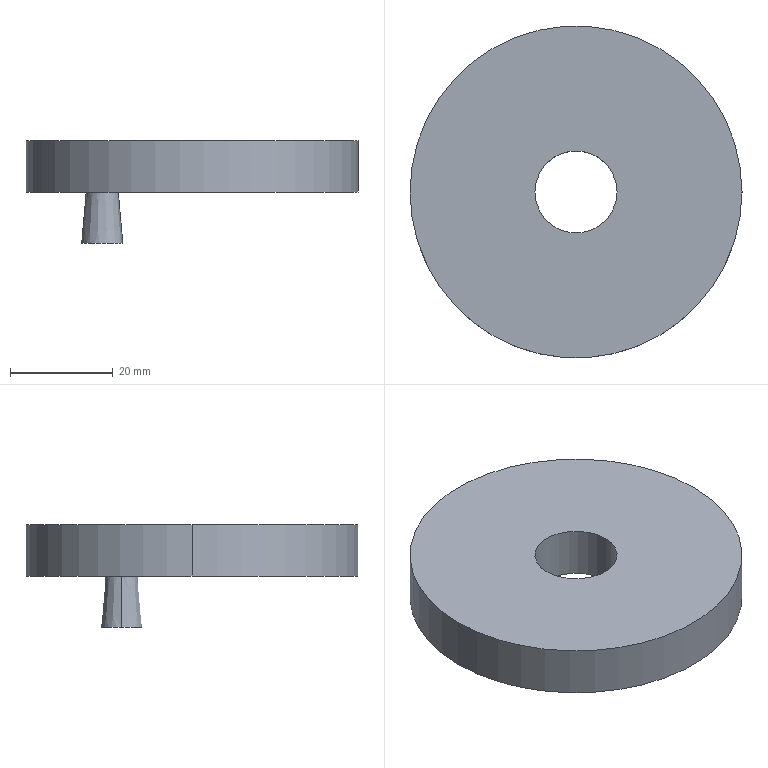Component | SolidWorks | RockerArm-1 | 1 solid | 9 faces | box 64.66 x 64.66 x 20 mm | volume 31223 mm3 | cylinder 4 | plane 3 | cone 2 | commonest cylinder face diameters 16 x2 64.655 x2
build123d program:
from build123d import *

# Parameters (mm, degrees)
SKETCH1_R           = 32.328
SKETCH1_R_2         = 8
BOSS_EXTRUDE1_DEPTH = 10
SKETCH2_R           = 3.13
BOSS_EXTRUDE2_DEPTH = 10
BOSS_EXTRUDE2_DRAFT = -5


with BuildPart() as part:
    # Sketch1 → Boss-Extrude1 (new body)
    with BuildSketch(Plane.XY):
        with Locations((0, -208.707)):
            Circle(SKETCH1_R)
        with Locations((0, -208.707)):
            Circle(SKETCH1_R_2, mode=Mode.SUBTRACT)
    extrude(amount=-BOSS_EXTRUDE1_DEPTH)


with BuildPart() as boss_extrude2_tool:
    # Sketch2 → Boss-Extrude2 (with draft: the straight prism first)
    with BuildSketch(Plane.XY):
        with Locations((17.482, -194.977)):
            Circle(SKETCH2_R)
    extrude(amount=BOSS_EXTRUDE2_DEPTH)
    # Boss-Extrude2: the draft: its side faces are tilted about the plane it starts from
    boss_extrude2_sides = [boss_extrude2_tool.faces().sort_by_distance(p)[0] for p in [
        (14.352, -194.977, 5),
    ]]
    draft(boss_extrude2_sides, Plane.XY, BOSS_EXTRUDE2_DRAFT)


with BuildPart() as part_1:
    add(part.part)

    # Boss-Extrude2: add boss_extrude2_tool
    add(boss_extrude2_tool.part)


solid = part_1.part

# Placed as in the assembly
solid = solid.moved(Location((0, 0, -657.565), (-180, 0, 180)))
STEP:
#1=COLOUR_RGB('',0.7922,0.8196,0.9333);
#2=FILL_AREA_STYLE_COLOUR('',#1);
#3=FILL_AREA_STYLE('',(#2));
#4=SURFACE_STYLE_FILL_AREA(#3);
#5=SURFACE_SIDE_STYLE('',(#4));
#6=SURFACE_STYLE_USAGE(.BOTH.,#5);
#7=PRESENTATION_STYLE_ASSIGNMENT((#6));
#8=CARTESIAN_POINT('',(-0.8115,-7.676,-25.888));
#9=VERTEX_POINT('',#8);
#10=CARTESIAN_POINT('',(-0.5651,-7.676,-25.888));
#11=VERTEX_POINT('',#10);
#12=CARTESIAN_POINT('',(-0.6883,-7.676,-25.888));
#13=DIRECTION('',(0.,0.,-1.));
#14=DIRECTION('',(-1.,0.,0.));
#15=AXIS2_PLACEMENT_3D('',#12,#13,#14);
#16=CIRCLE('',#15,0.1232);
#17=EDGE_CURVE('',#9,#11,#16,.T.);
#18=ORIENTED_EDGE('',*,*,#17,.T.);
#19=CARTESIAN_POINT('',(-0.5306,-7.676,-26.282));
#20=VERTEX_POINT('',#19);
#21=CARTESIAN_POINT('',(-0.5651,-7.676,-25.888));
#22=DIRECTION('',(0.08716,0.,-0.9962));
#23=VECTOR('',#22,39.37);
#24=LINE('',#21,#23);
#25=EDGE_CURVE('',#11,#20,#24,.T.);
#26=ORIENTED_EDGE('',*,*,#25,.T.);
#27=CARTESIAN_POINT('',(-0.8459,-7.676,-26.282));
#28=VERTEX_POINT('',#27);
#29=CARTESIAN_POINT('',(-0.6883,-7.676,-26.282));
#30=DIRECTION('',(0.,0.,-1.));
#31=DIRECTION('',(-1.,0.,0.));
#32=AXIS2_PLACEMENT_3D('',#29,#30,#31);
#33=CIRCLE('',#32,0.1577);
#34=EDGE_CURVE('',#28,#20,#33,.T.);
#35=ORIENTED_EDGE('',*,*,#34,.F.);
#36=CARTESIAN_POINT('',(-0.8115,-7.676,-25.888));
#37=DIRECTION('',(-0.08716,0.,-0.9962));
#38=VECTOR('',#37,39.37);
#39=LINE('',#36,#38);
#40=EDGE_CURVE('',#9,#28,#39,.T.);
#41=ORIENTED_EDGE('',*,*,#40,.F.);
#42=EDGE_LOOP('',(#18,#26,#35,#41));
#43=FACE_OUTER_BOUND('',#42,.T.);
#44=CARTESIAN_POINT('',(-0.6883,-7.676,-25.888));
#45=DIRECTION('',(0.,0.,-1.));
#46=DIRECTION('',(-1.,0.,0.));
#47=AXIS2_PLACEMENT_3D('',#44,#45,#46);
#48=CONICAL_SURFACE('',#47,0.1232,0.08727);
#49=ADVANCED_FACE('',(#43),#48,.T.);
#50=CARTESIAN_POINT('',(0.315,-8.217,-25.495));
#51=VERTEX_POINT('',#50);
#52=CARTESIAN_POINT('',(-0.315,-8.217,-25.495));
#53=VERTEX_POINT('',#52);
#54=CARTESIAN_POINT('',(0.,-8.217,-25.495));
#55=DIRECTION('',(0.,0.,-1.));
#56=DIRECTION('',(-1.,0.,0.));
#57=AXIS2_PLACEMENT_3D('',#54,#55,#56);
#58=CIRCLE('',#57,0.315);
#59=EDGE_CURVE('',#51,#53,#58,.T.);
#60=ORIENTED_EDGE('',*,*,#59,.F.);
#61=CARTESIAN_POINT('',(0.315,-8.217,-25.888));
#62=VERTEX_POINT('',#61);
#63=CARTESIAN_POINT('',(0.315,-8.217,-25.495));
#64=DIRECTION('',(0.,0.,-1.));
#65=VECTOR('',#64,39.37);
#66=LINE('',#63,#65);
#67=EDGE_CURVE('',#51,#62,#66,.T.);
#68=ORIENTED_EDGE('',*,*,#67,.T.);
#69=CARTESIAN_POINT('',(-0.315,-8.217,-25.888));
#70=VERTEX_POINT('',#69);
#71=CARTESIAN_POINT('',(0.,-8.217,-25.888));
#72=DIRECTION('',(0.,0.,-1.));
#73=DIRECTION('',(-1.,0.,0.));
#74=AXIS2_PLACEMENT_3D('',#71,#72,#73);
#75=CIRCLE('',#74,0.315);
#76=EDGE_CURVE('',#62,#70,#75,.T.);
#77=ORIENTED_EDGE('',*,*,#76,.T.);
#78=CARTESIAN_POINT('',(-0.315,-8.217,-25.495));
#79=DIRECTION('',(0.,0.,-1.));
#80=VECTOR('',#79,39.37);
#81=LINE('',#78,#80);
#82=EDGE_CURVE('',#53,#70,#81,.T.);
#83=ORIENTED_EDGE('',*,*,#82,.F.);
#84=EDGE_LOOP('',(#60,#68,#77,#83));
#85=FACE_OUTER_BOUND('',#84,.T.);
#86=CARTESIAN_POINT('',(0.,-8.217,-25.495));
#87=DIRECTION('',(0.,0.,-1.));
#88=DIRECTION('',(-1.,0.,0.));
#89=AXIS2_PLACEMENT_3D('',#86,#87,#88);
#90=CYLINDRICAL_SURFACE('',#89,0.315);
#91=ADVANCED_FACE('',(#85),#90,.F.);
#92=CARTESIAN_POINT('',(-1.273,-8.217,-25.495));
#93=VERTEX_POINT('',#92);
#94=CARTESIAN_POINT('',(1.273,-8.217,-25.495));
#95=VERTEX_POINT('',#94);
#96=CARTESIAN_POINT('',(0.,-8.217,-25.495));
#97=DIRECTION('',(0.,0.,-1.));
#98=DIRECTION('',(-1.,0.,0.));
#99=AXIS2_PLACEMENT_3D('',#96,#97,#98);
#100=CIRCLE('',#99,1.273);
#101=EDGE_CURVE('',#93,#95,#100,.T.);
#102=ORIENTED_EDGE('',*,*,#101,.T.);
#103=CARTESIAN_POINT('',(1.273,-8.217,-25.888));
#104=VERTEX_POINT('',#103);
#105=CARTESIAN_POINT('',(1.273,-8.217,-25.495));
#106=DIRECTION('',(0.,0.,-1.));
#107=VECTOR('',#106,39.37);
#108=LINE('',#105,#107);
#109=EDGE_CURVE('',#95,#104,#108,.T.);
#110=ORIENTED_EDGE('',*,*,#109,.T.);
#111=CARTESIAN_POINT('',(-1.273,-8.217,-25.888));
#112=VERTEX_POINT('',#111);
#113=CARTESIAN_POINT('',(0.,-8.217,-25.888));
#114=DIRECTION('',(0.,0.,-1.));
#115=DIRECTION('',(-1.,0.,0.));
#116=AXIS2_PLACEMENT_3D('',#113,#114,#115);
#117=CIRCLE('',#116,1.273);
#118=EDGE_CURVE('',#112,#104,#117,.T.);
#119=ORIENTED_EDGE('',*,*,#118,.F.);
#120=CARTESIAN_POINT('',(-1.273,-8.217,-25.495));
#121=DIRECTION('',(0.,0.,-1.));
#122=VECTOR('',#121,39.37);
#123=LINE('',#120,#122);
#124=EDGE_CURVE('',#93,#112,#123,.T.);
#125=ORIENTED_EDGE('',*,*,#124,.F.);
#126=EDGE_LOOP('',(#102,#110,#119,#125));
#127=FACE_OUTER_BOUND('',#126,.T.);
#128=CARTESIAN_POINT('',(0.,-8.217,-25.495));
#129=DIRECTION('',(0.,0.,-1.));
#130=DIRECTION('',(-1.,0.,0.));
#131=AXIS2_PLACEMENT_3D('',#128,#129,#130);
#132=CYLINDRICAL_SURFACE('',#131,1.273);
#133=ADVANCED_FACE('',(#127),#132,.T.);
#134=ORIENTED_EDGE('',*,*,#109,.F.);
#135=CARTESIAN_POINT('',(0.,-8.217,-25.495));
#136=DIRECTION('',(0.,0.,-1.));
#137=DIRECTION('',(-1.,0.,0.));
#138=AXIS2_PLACEMENT_3D('',#135,#136,#137);
#139=CIRCLE('',#138,1.273);
#140=EDGE_CURVE('',#95,#93,#139,.T.);
#141=ORIENTED_EDGE('',*,*,#140,.T.);
#142=ORIENTED_EDGE('',*,*,#124,.T.);
#143=CARTESIAN_POINT('',(0.,-8.217,-25.888));
#144=DIRECTION('',(0.,0.,-1.));
#145=DIRECTION('',(-1.,0.,0.));
#146=AXIS2_PLACEMENT_3D('',#143,#144,#145);
#147=CIRCLE('',#146,1.273);
#148=EDGE_CURVE('',#104,#112,#147,.T.);
#149=ORIENTED_EDGE('',*,*,#148,.F.);
#150=EDGE_LOOP('',(#134,#141,#142,#149));
#151=FACE_OUTER_BOUND('',#150,.T.);
#152=CARTESIAN_POINT('',(0.,-8.217,-25.495));
#153=DIRECTION('',(0.,0.,-1.));
#154=DIRECTION('',(-1.,0.,0.));
#155=AXIS2_PLACEMENT_3D('',#152,#153,#154);
#156=CYLINDRICAL_SURFACE('',#155,1.273);
#157=ADVANCED_FACE('',(#151),#156,.T.);
#158=CARTESIAN_POINT('',(0.,-8.217,-25.495));
#159=DIRECTION('',(0.,0.,-1.));
#160=DIRECTION('',(-1.,0.,0.));
#161=AXIS2_PLACEMENT_3D('',#158,#159,#160);
#162=CIRCLE('',#161,0.315);
#163=EDGE_CURVE('',#53,#51,#162,.T.);
#164=ORIENTED_EDGE('',*,*,#163,.T.);
#165=ORIENTED_EDGE('',*,*,#59,.T.);
#166=EDGE_LOOP('',(#164,#165));
#167=FACE_BOUND('',#166,.T.);
#168=ORIENTED_EDGE('',*,*,#101,.F.);
#169=ORIENTED_EDGE('',*,*,#140,.F.);
#170=EDGE_LOOP('',(#168,#169));
#171=FACE_OUTER_BOUND('',#170,.T.);
#172=CARTESIAN_POINT('',(0.,-8.217,-25.495));
#173=DIRECTION('',(0.,0.,-1.));
#174=DIRECTION('',(-1.,0.,0.));
#175=AXIS2_PLACEMENT_3D('',#172,#173,#174);
#176=PLANE('',#175);
#177=ADVANCED_FACE('',(#167,#171),#176,.F.);
#178=ORIENTED_EDGE('',*,*,#17,.F.);
#179=CARTESIAN_POINT('',(-0.6883,-7.676,-25.888));
#180=DIRECTION('',(0.,0.,-1.));
#181=DIRECTION('',(-1.,0.,0.));
#182=AXIS2_PLACEMENT_3D('',#179,#180,#181);
#183=CIRCLE('',#182,0.1232);
#184=EDGE_CURVE('',#11,#9,#183,.T.);
#185=ORIENTED_EDGE('',*,*,#184,.F.);
#186=EDGE_LOOP('',(#178,#185));
#187=FACE_BOUND('',#186,.T.);
#188=CARTESIAN_POINT('',(0.,-8.217,-25.888));
#189=DIRECTION('',(0.,0.,-1.));
#190=DIRECTION('',(-1.,0.,0.));
#191=AXIS2_PLACEMENT_3D('',#188,#189,#190);
#192=CIRCLE('',#191,0.315);
#193=EDGE_CURVE('',#70,#62,#192,.T.);
#194=ORIENTED_EDGE('',*,*,#193,.F.);
#195=ORIENTED_EDGE('',*,*,#76,.F.);
#196=EDGE_LOOP('',(#194,#195));
#197=FACE_BOUND('',#196,.T.);
#198=ORIENTED_EDGE('',*,*,#118,.T.);
#199=ORIENTED_EDGE('',*,*,#148,.T.);
#200=EDGE_LOOP('',(#198,#199));
#201=FACE_OUTER_BOUND('',#200,.T.);
#202=CARTESIAN_POINT('',(0.,-8.217,-25.888));
#203=DIRECTION('',(0.,0.,-1.));
#204=DIRECTION('',(-1.,0.,0.));
#205=AXIS2_PLACEMENT_3D('',#202,#203,#204);
#206=PLANE('',#205);
#207=ADVANCED_FACE('',(#187,#197,#201),#206,.T.);
#208=ORIENTED_EDGE('',*,*,#67,.F.);
#209=ORIENTED_EDGE('',*,*,#163,.F.);
#210=ORIENTED_EDGE('',*,*,#82,.T.);
#211=ORIENTED_EDGE('',*,*,#193,.T.);
#212=EDGE_LOOP('',(#208,#209,#210,#211));
#213=FACE_OUTER_BOUND('',#212,.T.);
#214=CARTESIAN_POINT('',(0.,-8.217,-25.495));
#215=DIRECTION('',(0.,0.,-1.));
#216=DIRECTION('',(-1.,0.,0.));
#217=AXIS2_PLACEMENT_3D('',#214,#215,#216);
#218=CYLINDRICAL_SURFACE('',#217,0.315);
#219=ADVANCED_FACE('',(#213),#218,.F.);
#220=ORIENTED_EDGE('',*,*,#25,.F.);
#221=ORIENTED_EDGE('',*,*,#184,.T.);
#222=ORIENTED_EDGE('',*,*,#40,.T.);
#223=CARTESIAN_POINT('',(-0.6883,-7.676,-26.282));
#224=DIRECTION('',(0.,0.,-1.));
#225=DIRECTION('',(-1.,0.,0.));
#226=AXIS2_PLACEMENT_3D('',#223,#224,#225);
#227=CIRCLE('',#226,0.1577);
#228=EDGE_CURVE('',#20,#28,#227,.T.);
#229=ORIENTED_EDGE('',*,*,#228,.F.);
#230=EDGE_LOOP('',(#220,#221,#222,#229));
#231=FACE_OUTER_BOUND('',#230,.T.);
#232=CARTESIAN_POINT('',(-0.6883,-7.676,-25.888));
#233=DIRECTION('',(0.,0.,-1.));
#234=DIRECTION('',(-1.,0.,0.));
#235=AXIS2_PLACEMENT_3D('',#232,#233,#234);
#236=CONICAL_SURFACE('',#235,0.1232,0.08727);
#237=ADVANCED_FACE('',(#231),#236,.T.);
#238=ORIENTED_EDGE('',*,*,#34,.T.);
#239=ORIENTED_EDGE('',*,*,#228,.T.);
#240=EDGE_LOOP('',(#238,#239));
#241=FACE_OUTER_BOUND('',#240,.T.);
#242=CARTESIAN_POINT('',(-0.6883,-7.676,-26.282));
#243=DIRECTION('',(0.,0.,-1.));
#244=DIRECTION('',(-1.,0.,0.));
#245=AXIS2_PLACEMENT_3D('',#242,#243,#244);
#246=PLANE('',#245);
#247=ADVANCED_FACE('',(#241),#246,.T.);
#248=CLOSED_SHELL('',(#49,#91,#133,#157,#177,#207,#219,#237,#247));
#249=MANIFOLD_SOLID_BREP('',#248);
#250=STYLED_ITEM('',(#7),#249);
#251=(LENGTH_UNIT()NAMED_UNIT(*)SI_UNIT($,.METRE.));
#252=LENGTH_MEASURE_WITH_UNIT(LENGTH_MEASURE(0.0254),#251);
#253=DIMENSIONAL_EXPONENTS(1.,0.,0.,0.,0.,0.,0.);
#254=(CONVERSION_BASED_UNIT('',#252)LENGTH_UNIT()NAMED_UNIT(#253));
#255=UNCERTAINTY_MEASURE_WITH_UNIT(LENGTH_MEASURE(0.00001),#254,'','');
#256=(NAMED_UNIT(*)PLANE_ANGLE_UNIT()SI_UNIT($,.RADIAN.));
#257=(NAMED_UNIT(*)SI_UNIT($,.STERADIAN.)SOLID_ANGLE_UNIT());
#258=(GEOMETRIC_REPRESENTATION_CONTEXT(3)GLOBAL_UNCERTAINTY_ASSIGNED_CONTEXT((#255))GLOBAL_UNIT_ASSIGNED_CONTEXT((#254,#256,#257))REPRESENTATION_CONTEXT('',''));
#259=MECHANICAL_DESIGN_GEOMETRIC_PRESENTATION_REPRESENTATION('',(#250),#258);
#260=CARTESIAN_POINT('',(0.,0.,0.));
#261=DIRECTION('',(0.,0.,1.));
#262=DIRECTION('',(1.,0.,0.));
#263=AXIS2_PLACEMENT_3D('',#260,#261,#262);
#264=(LENGTH_UNIT()NAMED_UNIT(*)SI_UNIT($,.METRE.));
#265=LENGTH_MEASURE_WITH_UNIT(LENGTH_MEASURE(0.0254),#264);
#266=DIMENSIONAL_EXPONENTS(1.,0.,0.,0.,0.,0.,0.);
#267=(CONVERSION_BASED_UNIT('',#265)LENGTH_UNIT()NAMED_UNIT(#266));
#268=UNCERTAINTY_MEASURE_WITH_UNIT(LENGTH_MEASURE(0.00001),#267,'','');
#269=(NAMED_UNIT(*)PLANE_ANGLE_UNIT()SI_UNIT($,.RADIAN.));
#270=(NAMED_UNIT(*)SI_UNIT($,.STERADIAN.)SOLID_ANGLE_UNIT());
#271=(GEOMETRIC_REPRESENTATION_CONTEXT(3)GLOBAL_UNCERTAINTY_ASSIGNED_CONTEXT((#268))GLOBAL_UNIT_ASSIGNED_CONTEXT((#267,#269,#270))REPRESENTATION_CONTEXT('',''));
#272=ADVANCED_BREP_SHAPE_REPRESENTATION('',(#249,#263),#271);
#273=PRESENTATION_LAYER_ASSIGNMENT('','',(#250));